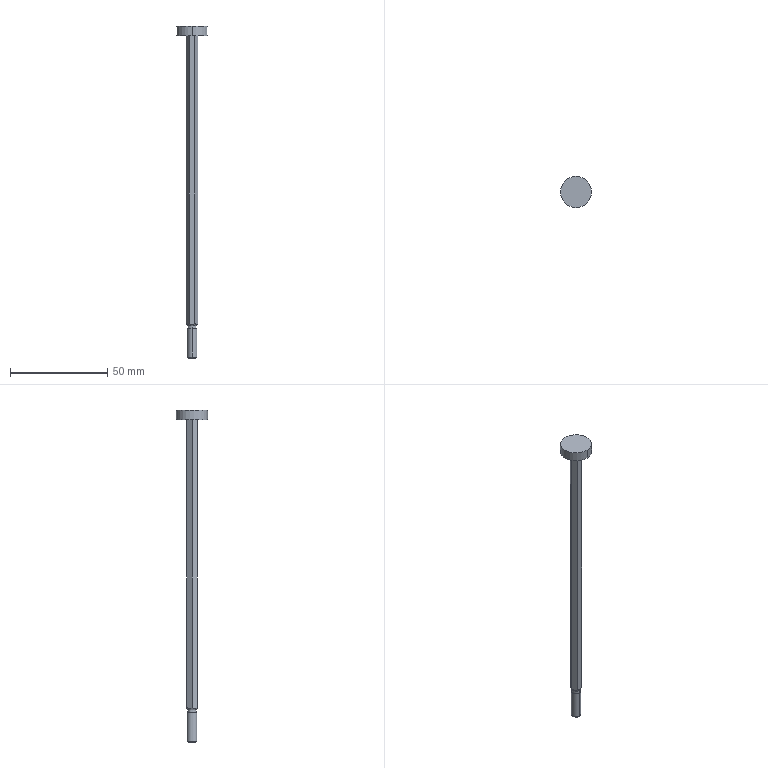Component | SolidWorks | F-YBCJ2RKA16-125_ROD-1 | 1 solid | 20 faces | box 16 x 16 x 170.5 mm | volume 4806 mm3 | plane 10 | cylinder 6 | cone 4 | commonest cylinder face diameters 16 x2 4.43 x2 5 x2
build123d program:
from build123d import *

# Parameters (mm, degrees)
SKETCH2_R          = 5.2
CUT_EXTRUDE1_DEPTH = 150.5


with BuildPart() as part:
    # Sketch1 → Revolve1 (revolve)
    with BuildSketch(Plane.XY, mode=Mode.PRIVATE) as revolve1_sk:
        Polygon((0, 0), (0, 2.01), (0.4905, 2.5), (15, 2.5), (15, 2.215), (16.5, 2.215), (17.864, 3.002), (165.5, 3.002), (165.5, 8), (170.5, 8), (170.5, 0), align=None)
    revolve(revolve1_sk.sketch.rotate(Axis((170.5, 0, 0), (-1, 0, 0)), 180), axis=Axis((170.5, 0, 0), (-1, 0, 0)))

    # Sketch2 → Cut-Extrude1 (cut)
    with BuildSketch(Plane(origin=(15, 0, 0), x_dir=(0, 0, -1), z_dir=(1, 0, 0))):
        Circle(SKETCH2_R)
        Polygon((-3.002, 0), (-1.501, -2.6), (1.501, -2.6), (3.002, 0), (1.501, 2.6), (-1.501, 2.6), align=None, mode=Mode.SUBTRACT)
    extrude(amount=CUT_EXTRUDE1_DEPTH, mode=Mode.SUBTRACT)


solid = part.part

# Placed as in the assembly
solid = solid.moved(Location((272.305, 302.175, 105.479), (0, -90, 0)))
STEP:
#1=COLOUR_RGB('',0.7922,0.8196,0.9333);
#2=FILL_AREA_STYLE_COLOUR('',#1);
#3=FILL_AREA_STYLE('',(#2));
#4=SURFACE_STYLE_FILL_AREA(#3);
#5=SURFACE_SIDE_STYLE('',(#4));
#6=SURFACE_STYLE_USAGE(.BOTH.,#5);
#7=PRESENTATION_STYLE_ASSIGNMENT((#6));
#8=CARTESIAN_POINT('',(10.721,11.582,10.865));
#9=VERTEX_POINT('',#8);
#10=CARTESIAN_POINT('',(10.721,12.212,10.865));
#11=VERTEX_POINT('',#10);
#12=CARTESIAN_POINT('',(10.721,11.897,10.865));
#13=DIRECTION('',(0.,-0.,-1.));
#14=DIRECTION('',(0.,-1.,0.));
#15=AXIS2_PLACEMENT_3D('',#12,#13,#14);
#16=CIRCLE('',#15,0.315);
#17=EDGE_CURVE('',#9,#11,#16,.T.);
#18=ORIENTED_EDGE('',*,*,#17,.T.);
#19=CARTESIAN_POINT('',(10.721,12.212,10.668));
#20=VERTEX_POINT('',#19);
#21=CARTESIAN_POINT('',(10.721,12.212,10.865));
#22=DIRECTION('',(0.,-0.,-1.));
#23=VECTOR('',#22,39.37);
#24=LINE('',#21,#23);
#25=EDGE_CURVE('',#11,#20,#24,.T.);
#26=ORIENTED_EDGE('',*,*,#25,.T.);
#27=CARTESIAN_POINT('',(10.721,11.582,10.668));
#28=VERTEX_POINT('',#27);
#29=CARTESIAN_POINT('',(10.721,11.897,10.668));
#30=DIRECTION('',(0.,-0.,-1.));
#31=DIRECTION('',(0.,-1.,0.));
#32=AXIS2_PLACEMENT_3D('',#29,#30,#31);
#33=CIRCLE('',#32,0.315);
#34=EDGE_CURVE('',#28,#20,#33,.T.);
#35=ORIENTED_EDGE('',*,*,#34,.F.);
#36=CARTESIAN_POINT('',(10.721,11.582,10.865));
#37=DIRECTION('',(0.,-0.,-1.));
#38=VECTOR('',#37,39.37);
#39=LINE('',#36,#38);
#40=EDGE_CURVE('',#9,#28,#39,.T.);
#41=ORIENTED_EDGE('',*,*,#40,.F.);
#42=EDGE_LOOP('',(#18,#26,#35,#41));
#43=FACE_OUTER_BOUND('',#42,.T.);
#44=CARTESIAN_POINT('',(10.721,11.897,10.865));
#45=DIRECTION('',(0.,-0.,-1.));
#46=DIRECTION('',(0.,-1.,0.));
#47=AXIS2_PLACEMENT_3D('',#44,#45,#46);
#48=CYLINDRICAL_SURFACE('',#47,0.315);
#49=ADVANCED_FACE('',(#43),#48,.T.);
#50=CARTESIAN_POINT('',(10.721,11.809,4.802));
#51=VERTEX_POINT('',#50);
#52=CARTESIAN_POINT('',(10.721,11.984,4.802));
#53=VERTEX_POINT('',#52);
#54=CARTESIAN_POINT('',(10.721,11.897,4.802));
#55=DIRECTION('',(0.,-0.,-1.));
#56=DIRECTION('',(0.,-1.,0.));
#57=AXIS2_PLACEMENT_3D('',#54,#55,#56);
#58=CIRCLE('',#57,0.0872);
#59=EDGE_CURVE('',#51,#53,#58,.T.);
#60=ORIENTED_EDGE('',*,*,#59,.F.);
#61=CARTESIAN_POINT('',(10.721,11.794,4.829));
#62=VERTEX_POINT('',#61);
#63=CARTESIAN_POINT('',(10.721,11.778,4.856));
#64=DIRECTION('',(-0.,-0.5,0.866));
#65=VECTOR('',#64,39.37);
#66=LINE('',#63,#65);
#67=EDGE_CURVE('',#51,#62,#66,.T.);
#68=ORIENTED_EDGE('',*,*,#67,.T.);
#69=CARTESIAN_POINT('',(10.662,11.794,4.856));
#70=VERTEX_POINT('',#69);
#71=CARTESIAN_POINT('',(10.721,11.794,4.829));
#72=CARTESIAN_POINT('',(10.71,11.794,4.829));
#73=CARTESIAN_POINT('',(10.699,11.794,4.832));
#74=CARTESIAN_POINT('',(10.679,11.794,4.842));
#75=CARTESIAN_POINT('',(10.67,11.794,4.849));
#76=CARTESIAN_POINT('',(10.662,11.794,4.856));
#77=B_SPLINE_CURVE_WITH_KNOTS('',3,(#71,#72,#73,#74,#75,#76),.UNSPECIFIED.,.F.,.F.,(4,2,4),(0.00333,0.004165,0.005),.UNSPECIFIED.);
#78=EDGE_CURVE('',#62,#70,#77,.T.);
#79=ORIENTED_EDGE('',*,*,#78,.T.);
#80=CARTESIAN_POINT('',(10.602,11.897,4.856));
#81=VERTEX_POINT('',#80);
#82=CARTESIAN_POINT('',(10.662,11.794,4.856));
#83=CARTESIAN_POINT('',(10.657,11.802,4.849));
#84=CARTESIAN_POINT('',(10.653,11.809,4.842));
#85=CARTESIAN_POINT('',(10.646,11.822,4.834));
#86=CARTESIAN_POINT('',(10.643,11.827,4.832));
#87=CARTESIAN_POINT('',(10.638,11.836,4.829));
#88=CARTESIAN_POINT('',(10.635,11.841,4.829));
#89=CARTESIAN_POINT('',(10.627,11.855,4.829));
#90=CARTESIAN_POINT('',(10.621,11.865,4.832));
#91=CARTESIAN_POINT('',(10.611,11.882,4.842));
#92=CARTESIAN_POINT('',(10.607,11.889,4.849));
#93=CARTESIAN_POINT('',(10.602,11.897,4.856));
#94=B_SPLINE_CURVE_WITH_KNOTS('',3,(#82,#83,#84,#85,#86,#87,#88,#89,#90,#91,#92,#93),.UNSPECIFIED.,.F.,.F.,(4,2,2,2,2,4),(0.0000003,0.0008398,0.00126,0.001679,0.002519,0.003358),.UNSPECIFIED.);
#95=EDGE_CURVE('',#70,#81,#94,.T.);
#96=ORIENTED_EDGE('',*,*,#95,.T.);
#97=CARTESIAN_POINT('',(10.662,11.999,4.856));
#98=VERTEX_POINT('',#97);
#99=CARTESIAN_POINT('',(10.602,11.897,4.856));
#100=CARTESIAN_POINT('',(10.607,11.904,4.849));
#101=CARTESIAN_POINT('',(10.611,11.912,4.842));
#102=CARTESIAN_POINT('',(10.618,11.924,4.834));
#103=CARTESIAN_POINT('',(10.621,11.929,4.832));
#104=CARTESIAN_POINT('',(10.626,11.938,4.829));
#105=CARTESIAN_POINT('',(10.629,11.943,4.829));
#106=CARTESIAN_POINT('',(10.638,11.957,4.829));
#107=CARTESIAN_POINT('',(10.643,11.967,4.832));
#108=CARTESIAN_POINT('',(10.653,11.984,4.842));
#109=CARTESIAN_POINT('',(10.657,11.992,4.849));
#110=CARTESIAN_POINT('',(10.662,11.999,4.856));
#111=B_SPLINE_CURVE_WITH_KNOTS('',3,(#99,#100,#101,#102,#103,#104,#105,#106,#107,#108,#109,#110),.UNSPECIFIED.,.F.,.F.,(4,2,2,2,2,4),(0.0000003,0.0008398,0.00126,0.001679,0.002519,0.003358),.UNSPECIFIED.);
#112=EDGE_CURVE('',#81,#98,#111,.T.);
#113=ORIENTED_EDGE('',*,*,#112,.T.);
#114=CARTESIAN_POINT('',(10.721,11.999,4.829));
#115=VERTEX_POINT('',#114);
#116=CARTESIAN_POINT('',(10.662,11.999,4.856));
#117=CARTESIAN_POINT('',(10.67,11.999,4.849));
#118=CARTESIAN_POINT('',(10.679,11.999,4.842));
#119=CARTESIAN_POINT('',(10.699,11.999,4.832));
#120=CARTESIAN_POINT('',(10.71,11.999,4.829));
#121=CARTESIAN_POINT('',(10.721,11.999,4.829));
#122=B_SPLINE_CURVE_WITH_KNOTS('',3,(#116,#117,#118,#119,#120,#121),.UNSPECIFIED.,.F.,.F.,(4,2,4),(0.003237,0.004069,0.004901),.UNSPECIFIED.);
#123=EDGE_CURVE('',#98,#115,#122,.T.);
#124=ORIENTED_EDGE('',*,*,#123,.T.);
#125=CARTESIAN_POINT('',(10.721,12.015,4.856));
#126=DIRECTION('',(-0.,0.5,0.866));
#127=VECTOR('',#126,39.37);
#128=LINE('',#125,#127);
#129=EDGE_CURVE('',#53,#115,#128,.T.);
#130=ORIENTED_EDGE('',*,*,#129,.F.);
#131=EDGE_LOOP('',(#60,#68,#79,#96,#113,#124,#130));
#132=FACE_OUTER_BOUND('',#131,.T.);
#133=CARTESIAN_POINT('',(10.721,11.897,4.856));
#134=DIRECTION('',(-0.,0.,1.));
#135=DIRECTION('',(0.,1.,0.));
#136=AXIS2_PLACEMENT_3D('',#133,#134,#135);
#137=CONICAL_SURFACE('',#136,0.1182,0.5236);
#138=ADVANCED_FACE('',(#132),#137,.T.);
#139=ORIENTED_EDGE('',*,*,#59,.T.);
#140=CARTESIAN_POINT('',(10.721,11.984,4.743));
#141=VERTEX_POINT('',#140);
#142=CARTESIAN_POINT('',(10.721,11.984,10.865));
#143=DIRECTION('',(0.,-0.,-1.));
#144=VECTOR('',#143,39.37);
#145=LINE('',#142,#144);
#146=EDGE_CURVE('',#53,#141,#145,.T.);
#147=ORIENTED_EDGE('',*,*,#146,.T.);
#148=CARTESIAN_POINT('',(10.721,11.809,4.743));
#149=VERTEX_POINT('',#148);
#150=CARTESIAN_POINT('',(10.721,11.897,4.743));
#151=DIRECTION('',(0.,-0.,-1.));
#152=DIRECTION('',(0.,-1.,0.));
#153=AXIS2_PLACEMENT_3D('',#150,#151,#152);
#154=CIRCLE('',#153,0.0872);
#155=EDGE_CURVE('',#149,#141,#154,.T.);
#156=ORIENTED_EDGE('',*,*,#155,.F.);
#157=CARTESIAN_POINT('',(10.721,11.809,10.865));
#158=DIRECTION('',(0.,-0.,-1.));
#159=VECTOR('',#158,39.37);
#160=LINE('',#157,#159);
#161=EDGE_CURVE('',#51,#149,#160,.T.);
#162=ORIENTED_EDGE('',*,*,#161,.F.);
#163=EDGE_LOOP('',(#139,#147,#156,#162));
#164=FACE_OUTER_BOUND('',#163,.T.);
#165=CARTESIAN_POINT('',(10.721,11.897,10.865));
#166=DIRECTION('',(0.,-0.,-1.));
#167=DIRECTION('',(0.,-1.,0.));
#168=AXIS2_PLACEMENT_3D('',#165,#166,#167);
#169=CYLINDRICAL_SURFACE('',#168,0.0872);
#170=ADVANCED_FACE('',(#164),#169,.T.);
#171=CARTESIAN_POINT('',(10.721,11.798,4.743));
#172=VERTEX_POINT('',#171);
#173=CARTESIAN_POINT('',(10.721,11.995,4.743));
#174=VERTEX_POINT('',#173);
#175=CARTESIAN_POINT('',(10.721,11.897,4.743));
#176=DIRECTION('',(0.,-0.,-1.));
#177=DIRECTION('',(0.,-1.,0.));
#178=AXIS2_PLACEMENT_3D('',#175,#176,#177);
#179=CIRCLE('',#178,0.09843);
#180=EDGE_CURVE('',#172,#174,#179,.T.);
#181=ORIENTED_EDGE('',*,*,#180,.T.);
#182=CARTESIAN_POINT('',(10.721,11.995,4.172));
#183=VERTEX_POINT('',#182);
#184=CARTESIAN_POINT('',(10.721,11.995,10.865));
#185=DIRECTION('',(0.,-0.,-1.));
#186=VECTOR('',#185,39.37);
#187=LINE('',#184,#186);
#188=EDGE_CURVE('',#174,#183,#187,.T.);
#189=ORIENTED_EDGE('',*,*,#188,.T.);
#190=CARTESIAN_POINT('',(10.721,11.798,4.172));
#191=VERTEX_POINT('',#190);
#192=CARTESIAN_POINT('',(10.721,11.897,4.172));
#193=DIRECTION('',(0.,-0.,-1.));
#194=DIRECTION('',(0.,-1.,0.));
#195=AXIS2_PLACEMENT_3D('',#192,#193,#194);
#196=CIRCLE('',#195,0.09843);
#197=EDGE_CURVE('',#191,#183,#196,.T.);
#198=ORIENTED_EDGE('',*,*,#197,.F.);
#199=CARTESIAN_POINT('',(10.721,11.798,10.865));
#200=DIRECTION('',(0.,-0.,-1.));
#201=VECTOR('',#200,39.37);
#202=LINE('',#199,#201);
#203=EDGE_CURVE('',#172,#191,#202,.T.);
#204=ORIENTED_EDGE('',*,*,#203,.F.);
#205=EDGE_LOOP('',(#181,#189,#198,#204));
#206=FACE_OUTER_BOUND('',#205,.T.);
#207=CARTESIAN_POINT('',(10.721,11.897,10.865));
#208=DIRECTION('',(0.,-0.,-1.));
#209=DIRECTION('',(0.,-1.,0.));
#210=AXIS2_PLACEMENT_3D('',#207,#208,#209);
#211=CYLINDRICAL_SURFACE('',#210,0.09843);
#212=ADVANCED_FACE('',(#206),#211,.T.);
#213=CARTESIAN_POINT('',(10.721,11.818,4.153));
#214=VERTEX_POINT('',#213);
#215=CARTESIAN_POINT('',(10.721,11.976,4.153));
#216=VERTEX_POINT('',#215);
#217=CARTESIAN_POINT('',(10.721,11.897,4.153));
#218=DIRECTION('',(0.,-0.,-1.));
#219=DIRECTION('',(0.,-1.,0.));
#220=AXIS2_PLACEMENT_3D('',#217,#218,#219);
#221=CIRCLE('',#220,0.07911);
#222=EDGE_CURVE('',#214,#216,#221,.T.);
#223=ORIENTED_EDGE('',*,*,#222,.F.);
#224=CARTESIAN_POINT('',(10.721,11.798,4.172));
#225=DIRECTION('',(-0.,-0.7071,0.7071));
#226=VECTOR('',#225,39.37);
#227=LINE('',#224,#226);
#228=EDGE_CURVE('',#214,#191,#227,.T.);
#229=ORIENTED_EDGE('',*,*,#228,.T.);
#230=ORIENTED_EDGE('',*,*,#197,.T.);
#231=CARTESIAN_POINT('',(10.721,11.995,4.172));
#232=DIRECTION('',(-0.,0.7071,0.7071));
#233=VECTOR('',#232,39.37);
#234=LINE('',#231,#233);
#235=EDGE_CURVE('',#216,#183,#234,.T.);
#236=ORIENTED_EDGE('',*,*,#235,.F.);
#237=EDGE_LOOP('',(#223,#229,#230,#236));
#238=FACE_OUTER_BOUND('',#237,.T.);
#239=CARTESIAN_POINT('',(10.721,11.897,4.172));
#240=DIRECTION('',(-0.,0.,1.));
#241=DIRECTION('',(0.,1.,0.));
#242=AXIS2_PLACEMENT_3D('',#239,#240,#241);
#243=CONICAL_SURFACE('',#242,0.09843,0.7854);
#244=ADVANCED_FACE('',(#238),#243,.T.);
#245=CARTESIAN_POINT('',(10.721,11.897,4.153));
#246=DIRECTION('',(0.,-0.,-1.));
#247=DIRECTION('',(0.,-1.,0.));
#248=AXIS2_PLACEMENT_3D('',#245,#246,#247);
#249=CIRCLE('',#248,0.07911);
#250=EDGE_CURVE('',#216,#214,#249,.T.);
#251=ORIENTED_EDGE('',*,*,#250,.T.);
#252=ORIENTED_EDGE('',*,*,#222,.T.);
#253=EDGE_LOOP('',(#251,#252));
#254=FACE_OUTER_BOUND('',#253,.T.);
#255=CARTESIAN_POINT('',(10.721,11.897,4.153));
#256=DIRECTION('',(-0.,0.,1.));
#257=DIRECTION('',(0.,1.,-0.));
#258=AXIS2_PLACEMENT_3D('',#255,#256,#257);
#259=PLANE('',#258);
#260=ADVANCED_FACE('',(#254),#259,.F.);
#261=ORIENTED_EDGE('',*,*,#228,.F.);
#262=ORIENTED_EDGE('',*,*,#250,.F.);
#263=ORIENTED_EDGE('',*,*,#235,.T.);
#264=CARTESIAN_POINT('',(10.721,11.897,4.172));
#265=DIRECTION('',(0.,-0.,-1.));
#266=DIRECTION('',(0.,-1.,0.));
#267=AXIS2_PLACEMENT_3D('',#264,#265,#266);
#268=CIRCLE('',#267,0.09843);
#269=EDGE_CURVE('',#183,#191,#268,.T.);
#270=ORIENTED_EDGE('',*,*,#269,.T.);
#271=EDGE_LOOP('',(#261,#262,#263,#270));
#272=FACE_OUTER_BOUND('',#271,.T.);
#273=CARTESIAN_POINT('',(10.721,11.897,4.172));
#274=DIRECTION('',(-0.,0.,1.));
#275=DIRECTION('',(0.,1.,0.));
#276=AXIS2_PLACEMENT_3D('',#273,#274,#275);
#277=CONICAL_SURFACE('',#276,0.09843,0.7854);
#278=ADVANCED_FACE('',(#272),#277,.T.);
#279=ORIENTED_EDGE('',*,*,#188,.F.);
#280=CARTESIAN_POINT('',(10.721,11.897,4.743));
#281=DIRECTION('',(0.,-0.,-1.));
#282=DIRECTION('',(0.,-1.,0.));
#283=AXIS2_PLACEMENT_3D('',#280,#281,#282);
#284=CIRCLE('',#283,0.09843);
#285=EDGE_CURVE('',#174,#172,#284,.T.);
#286=ORIENTED_EDGE('',*,*,#285,.T.);
#287=ORIENTED_EDGE('',*,*,#203,.T.);
#288=ORIENTED_EDGE('',*,*,#269,.F.);
#289=EDGE_LOOP('',(#279,#286,#287,#288));
#290=FACE_OUTER_BOUND('',#289,.T.);
#291=CARTESIAN_POINT('',(10.721,11.897,10.865));
#292=DIRECTION('',(0.,-0.,-1.));
#293=DIRECTION('',(0.,-1.,0.));
#294=AXIS2_PLACEMENT_3D('',#291,#292,#293);
#295=CYLINDRICAL_SURFACE('',#294,0.09843);
#296=ADVANCED_FACE('',(#290),#295,.T.);
#297=ORIENTED_EDGE('',*,*,#180,.F.);
#298=ORIENTED_EDGE('',*,*,#285,.F.);
#299=EDGE_LOOP('',(#297,#298));
#300=FACE_OUTER_BOUND('',#299,.T.);
#301=ORIENTED_EDGE('',*,*,#155,.T.);
#302=CARTESIAN_POINT('',(10.721,11.897,4.743));
#303=DIRECTION('',(0.,-0.,-1.));
#304=DIRECTION('',(0.,-1.,0.));
#305=AXIS2_PLACEMENT_3D('',#302,#303,#304);
#306=CIRCLE('',#305,0.0872);
#307=EDGE_CURVE('',#141,#149,#306,.T.);
#308=ORIENTED_EDGE('',*,*,#307,.T.);
#309=EDGE_LOOP('',(#301,#308));
#310=FACE_BOUND('',#309,.T.);
#311=CARTESIAN_POINT('',(10.721,11.995,4.743));
#312=DIRECTION('',(0.,-0.,-1.));
#313=DIRECTION('',(-0.,-1.,0.));
#314=AXIS2_PLACEMENT_3D('',#311,#312,#313);
#315=PLANE('',#314);
#316=ADVANCED_FACE('',(#300,#310),#315,.F.);
#317=ORIENTED_EDGE('',*,*,#146,.F.);
#318=CARTESIAN_POINT('',(10.721,11.897,4.802));
#319=DIRECTION('',(0.,-0.,-1.));
#320=DIRECTION('',(0.,-1.,0.));
#321=AXIS2_PLACEMENT_3D('',#318,#319,#320);
#322=CIRCLE('',#321,0.0872);
#323=EDGE_CURVE('',#53,#51,#322,.T.);
#324=ORIENTED_EDGE('',*,*,#323,.T.);
#325=ORIENTED_EDGE('',*,*,#161,.T.);
#326=ORIENTED_EDGE('',*,*,#307,.F.);
#327=EDGE_LOOP('',(#317,#324,#325,#326));
#328=FACE_OUTER_BOUND('',#327,.T.);
#329=CARTESIAN_POINT('',(10.721,11.897,10.865));
#330=DIRECTION('',(0.,-0.,-1.));
#331=DIRECTION('',(0.,-1.,0.));
#332=AXIS2_PLACEMENT_3D('',#329,#330,#331);
#333=CYLINDRICAL_SURFACE('',#332,0.0872);
#334=ADVANCED_FACE('',(#328),#333,.T.);
#335=ORIENTED_EDGE('',*,*,#67,.F.);
#336=ORIENTED_EDGE('',*,*,#323,.F.);
#337=ORIENTED_EDGE('',*,*,#129,.T.);
#338=CARTESIAN_POINT('',(10.78,11.999,4.856));
#339=VERTEX_POINT('',#338);
#340=CARTESIAN_POINT('',(10.721,11.999,4.829));
#341=CARTESIAN_POINT('',(10.732,11.999,4.829));
#342=CARTESIAN_POINT('',(10.743,11.999,4.832));
#343=CARTESIAN_POINT('',(10.762,11.999,4.842));
#344=CARTESIAN_POINT('',(10.771,11.999,4.849));
#345=CARTESIAN_POINT('',(10.78,11.999,4.856));
#346=B_SPLINE_CURVE_WITH_KNOTS('',3,(#340,#341,#342,#343,#344,#345),.UNSPECIFIED.,.F.,.F.,(4,2,4),(0.004901,0.005734,0.006567),.UNSPECIFIED.);
#347=EDGE_CURVE('',#115,#339,#346,.T.);
#348=ORIENTED_EDGE('',*,*,#347,.T.);
#349=CARTESIAN_POINT('',(10.839,11.897,4.856));
#350=VERTEX_POINT('',#349);
#351=CARTESIAN_POINT('',(10.78,11.999,4.856));
#352=CARTESIAN_POINT('',(10.784,11.992,4.849));
#353=CARTESIAN_POINT('',(10.788,11.984,4.842));
#354=CARTESIAN_POINT('',(10.796,11.971,4.834));
#355=CARTESIAN_POINT('',(10.798,11.967,4.832));
#356=CARTESIAN_POINT('',(10.804,11.958,4.829));
#357=CARTESIAN_POINT('',(10.807,11.953,4.829));
#358=CARTESIAN_POINT('',(10.815,11.938,4.829));
#359=CARTESIAN_POINT('',(10.82,11.929,4.832));
#360=CARTESIAN_POINT('',(10.83,11.912,4.842));
#361=CARTESIAN_POINT('',(10.835,11.904,4.849));
#362=CARTESIAN_POINT('',(10.839,11.897,4.856));
#363=B_SPLINE_CURVE_WITH_KNOTS('',3,(#351,#352,#353,#354,#355,#356,#357,#358,#359,#360,#361,#362),.UNSPECIFIED.,.F.,.F.,(4,2,2,2,2,4),(0.0000003,0.0008398,0.00126,0.001679,0.002519,0.003358),.UNSPECIFIED.);
#364=EDGE_CURVE('',#339,#350,#363,.T.);
#365=ORIENTED_EDGE('',*,*,#364,.T.);
#366=CARTESIAN_POINT('',(10.78,11.794,4.856));
#367=VERTEX_POINT('',#366);
#368=CARTESIAN_POINT('',(10.839,11.897,4.856));
#369=CARTESIAN_POINT('',(10.835,11.889,4.849));
#370=CARTESIAN_POINT('',(10.83,11.882,4.842));
#371=CARTESIAN_POINT('',(10.823,11.869,4.834));
#372=CARTESIAN_POINT('',(10.82,11.864,4.832));
#373=CARTESIAN_POINT('',(10.815,11.855,4.829));
#374=CARTESIAN_POINT('',(10.812,11.85,4.829));
#375=CARTESIAN_POINT('',(10.804,11.836,4.829));
#376=CARTESIAN_POINT('',(10.798,11.826,4.832));
#377=CARTESIAN_POINT('',(10.789,11.809,4.842));
#378=CARTESIAN_POINT('',(10.784,11.802,4.849));
#379=CARTESIAN_POINT('',(10.78,11.794,4.856));
#380=B_SPLINE_CURVE_WITH_KNOTS('',3,(#368,#369,#370,#371,#372,#373,#374,#375,#376,#377,#378,#379),.UNSPECIFIED.,.F.,.F.,(4,2,2,2,2,4),(0.0000003,0.0008398,0.00126,0.001679,0.002519,0.003358),.UNSPECIFIED.);
#381=EDGE_CURVE('',#350,#367,#380,.T.);
#382=ORIENTED_EDGE('',*,*,#381,.T.);
#383=CARTESIAN_POINT('',(10.78,11.794,4.856));
#384=CARTESIAN_POINT('',(10.771,11.794,4.849));
#385=CARTESIAN_POINT('',(10.762,11.794,4.842));
#386=CARTESIAN_POINT('',(10.743,11.794,4.832));
#387=CARTESIAN_POINT('',(10.732,11.794,4.829));
#388=CARTESIAN_POINT('',(10.721,11.794,4.829));
#389=B_SPLINE_CURVE_WITH_KNOTS('',3,(#383,#384,#385,#386,#387,#388),.UNSPECIFIED.,.F.,.F.,(4,2,4),(0.001658,0.002494,0.00333),.UNSPECIFIED.);
#390=EDGE_CURVE('',#367,#62,#389,.T.);
#391=ORIENTED_EDGE('',*,*,#390,.T.);
#392=EDGE_LOOP('',(#335,#336,#337,#348,#365,#382,#391));
#393=FACE_OUTER_BOUND('',#392,.T.);
#394=CARTESIAN_POINT('',(10.721,11.897,4.856));
#395=DIRECTION('',(-0.,0.,1.));
#396=DIRECTION('',(0.,1.,0.));
#397=AXIS2_PLACEMENT_3D('',#394,#395,#396);
#398=CONICAL_SURFACE('',#397,0.1182,0.5236);
#399=ADVANCED_FACE('',(#393),#398,.T.);
#400=CARTESIAN_POINT('',(10.602,11.897,10.668));
#401=VERTEX_POINT('',#400);
#402=CARTESIAN_POINT('',(10.602,11.897,10.668));
#403=DIRECTION('',(0.,0.,-1.));
#404=VECTOR('',#403,39.37);
#405=LINE('',#402,#404);
#406=EDGE_CURVE('',#401,#81,#405,.T.);
#407=ORIENTED_EDGE('',*,*,#406,.F.);
#408=CARTESIAN_POINT('',(10.662,11.999,10.668));
#409=VERTEX_POINT('',#408);
#410=CARTESIAN_POINT('',(10.662,11.999,10.668));
#411=DIRECTION('',(-0.5,-0.866,-0.));
#412=VECTOR('',#411,39.37);
#413=LINE('',#410,#412);
#414=EDGE_CURVE('',#409,#401,#413,.T.);
#415=ORIENTED_EDGE('',*,*,#414,.F.);
#416=CARTESIAN_POINT('',(10.662,11.999,10.668));
#417=DIRECTION('',(0.,0.,-1.));
#418=VECTOR('',#417,39.37);
#419=LINE('',#416,#418);
#420=EDGE_CURVE('',#409,#98,#419,.T.);
#421=ORIENTED_EDGE('',*,*,#420,.T.);
#422=ORIENTED_EDGE('',*,*,#112,.F.);
#423=EDGE_LOOP('',(#407,#415,#421,#422));
#424=FACE_OUTER_BOUND('',#423,.T.);
#425=CARTESIAN_POINT('',(10.662,11.999,10.668));
#426=DIRECTION('',(0.866,-0.5,0.));
#427=DIRECTION('',(0.5,0.866,0.));
#428=AXIS2_PLACEMENT_3D('',#425,#426,#427);
#429=PLANE('',#428);
#430=ADVANCED_FACE('',(#424),#429,.F.);
#431=CARTESIAN_POINT('',(10.662,11.794,10.668));
#432=VERTEX_POINT('',#431);
#433=CARTESIAN_POINT('',(10.662,11.794,10.668));
#434=DIRECTION('',(0.,0.,-1.));
#435=VECTOR('',#434,39.37);
#436=LINE('',#433,#435);
#437=EDGE_CURVE('',#432,#70,#436,.T.);
#438=ORIENTED_EDGE('',*,*,#437,.F.);
#439=CARTESIAN_POINT('',(10.602,11.897,10.668));
#440=DIRECTION('',(0.5,-0.866,0.));
#441=VECTOR('',#440,39.37);
#442=LINE('',#439,#441);
#443=EDGE_CURVE('',#401,#432,#442,.T.);
#444=ORIENTED_EDGE('',*,*,#443,.F.);
#445=ORIENTED_EDGE('',*,*,#406,.T.);
#446=ORIENTED_EDGE('',*,*,#95,.F.);
#447=EDGE_LOOP('',(#438,#444,#445,#446));
#448=FACE_OUTER_BOUND('',#447,.T.);
#449=CARTESIAN_POINT('',(10.602,11.897,10.668));
#450=DIRECTION('',(0.866,0.5,0.));
#451=DIRECTION('',(-0.5,0.866,-0.));
#452=AXIS2_PLACEMENT_3D('',#449,#450,#451);
#453=PLANE('',#452);
#454=ADVANCED_FACE('',(#448),#453,.F.);
#455=CARTESIAN_POINT('',(10.78,11.794,10.668));
#456=VERTEX_POINT('',#455);
#457=CARTESIAN_POINT('',(10.78,11.794,10.668));
#458=DIRECTION('',(0.,0.,-1.));
#459=VECTOR('',#458,39.37);
#460=LINE('',#457,#459);
#461=EDGE_CURVE('',#456,#367,#460,.T.);
#462=ORIENTED_EDGE('',*,*,#461,.F.);
#463=CARTESIAN_POINT('',(10.662,11.794,10.668));
#464=DIRECTION('',(1.,-0.,0.));
#465=VECTOR('',#464,39.37);
#466=LINE('',#463,#465);
#467=EDGE_CURVE('',#432,#456,#466,.T.);
#468=ORIENTED_EDGE('',*,*,#467,.F.);
#469=ORIENTED_EDGE('',*,*,#437,.T.);
#470=ORIENTED_EDGE('',*,*,#78,.F.);
#471=ORIENTED_EDGE('',*,*,#390,.F.);
#472=EDGE_LOOP('',(#462,#468,#469,#470,#471));
#473=FACE_OUTER_BOUND('',#472,.T.);
#474=CARTESIAN_POINT('',(10.662,11.794,10.668));
#475=DIRECTION('',(0.,1.,0.));
#476=DIRECTION('',(-1.,0.,-0.));
#477=AXIS2_PLACEMENT_3D('',#474,#475,#476);
#478=PLANE('',#477);
#479=ADVANCED_FACE('',(#473),#478,.F.);
#480=CARTESIAN_POINT('',(10.839,11.897,10.668));
#481=VERTEX_POINT('',#480);
#482=CARTESIAN_POINT('',(10.839,11.897,10.668));
#483=DIRECTION('',(0.,0.,-1.));
#484=VECTOR('',#483,39.37);
#485=LINE('',#482,#484);
#486=EDGE_CURVE('',#481,#350,#485,.T.);
#487=ORIENTED_EDGE('',*,*,#486,.F.);
#488=CARTESIAN_POINT('',(10.78,11.794,10.668));
#489=DIRECTION('',(0.5,0.866,0.));
#490=VECTOR('',#489,39.37);
#491=LINE('',#488,#490);
#492=EDGE_CURVE('',#456,#481,#491,.T.);
#493=ORIENTED_EDGE('',*,*,#492,.F.);
#494=ORIENTED_EDGE('',*,*,#461,.T.);
#495=ORIENTED_EDGE('',*,*,#381,.F.);
#496=EDGE_LOOP('',(#487,#493,#494,#495));
#497=FACE_OUTER_BOUND('',#496,.T.);
#498=CARTESIAN_POINT('',(10.78,11.794,10.668));
#499=DIRECTION('',(-0.866,0.5,-0.));
#500=DIRECTION('',(-0.5,-0.866,-0.));
#501=AXIS2_PLACEMENT_3D('',#498,#499,#500);
#502=PLANE('',#501);
#503=ADVANCED_FACE('',(#497),#502,.F.);
#504=CARTESIAN_POINT('',(10.78,11.999,10.668));
#505=VERTEX_POINT('',#504);
#506=CARTESIAN_POINT('',(10.78,11.999,10.668));
#507=DIRECTION('',(0.,0.,-1.));
#508=VECTOR('',#507,39.37);
#509=LINE('',#506,#508);
#510=EDGE_CURVE('',#505,#339,#509,.T.);
#511=ORIENTED_EDGE('',*,*,#510,.F.);
#512=CARTESIAN_POINT('',(10.839,11.897,10.668));
#513=DIRECTION('',(-0.5,0.866,-0.));
#514=VECTOR('',#513,39.37);
#515=LINE('',#512,#514);
#516=EDGE_CURVE('',#481,#505,#515,.T.);
#517=ORIENTED_EDGE('',*,*,#516,.F.);
#518=ORIENTED_EDGE('',*,*,#486,.T.);
#519=ORIENTED_EDGE('',*,*,#364,.F.);
#520=EDGE_LOOP('',(#511,#517,#518,#519));
#521=FACE_OUTER_BOUND('',#520,.T.);
#522=CARTESIAN_POINT('',(10.839,11.897,10.668));
#523=DIRECTION('',(-0.866,-0.5,-0.));
#524=DIRECTION('',(0.5,-0.866,0.));
#525=AXIS2_PLACEMENT_3D('',#522,#523,#524);
#526=PLANE('',#525);
#527=ADVANCED_FACE('',(#521),#526,.F.);
#528=ORIENTED_EDGE('',*,*,#420,.F.);
#529=CARTESIAN_POINT('',(10.78,11.999,10.668));
#530=DIRECTION('',(-1.,0.,-0.));
#531=VECTOR('',#530,39.37);
#532=LINE('',#529,#531);
#533=EDGE_CURVE('',#505,#409,#532,.T.);
#534=ORIENTED_EDGE('',*,*,#533,.F.);
#535=ORIENTED_EDGE('',*,*,#510,.T.);
#536=ORIENTED_EDGE('',*,*,#347,.F.);
#537=ORIENTED_EDGE('',*,*,#123,.F.);
#538=EDGE_LOOP('',(#528,#534,#535,#536,#537));
#539=FACE_OUTER_BOUND('',#538,.T.);
#540=CARTESIAN_POINT('',(10.78,11.999,10.668));
#541=DIRECTION('',(-0.,-1.,-0.));
#542=DIRECTION('',(1.,-0.,0.));
#543=AXIS2_PLACEMENT_3D('',#540,#541,#542);
#544=PLANE('',#543);
#545=ADVANCED_FACE('',(#539),#544,.F.);
#546=ORIENTED_EDGE('',*,*,#17,.F.);
#547=CARTESIAN_POINT('',(10.721,11.897,10.865));
#548=DIRECTION('',(0.,-0.,-1.));
#549=DIRECTION('',(0.,-1.,0.));
#550=AXIS2_PLACEMENT_3D('',#547,#548,#549);
#551=CIRCLE('',#550,0.315);
#552=EDGE_CURVE('',#11,#9,#551,.T.);
#553=ORIENTED_EDGE('',*,*,#552,.F.);
#554=EDGE_LOOP('',(#546,#553));
#555=FACE_OUTER_BOUND('',#554,.T.);
#556=CARTESIAN_POINT('',(10.721,12.212,10.865));
#557=DIRECTION('',(0.,-0.,-1.));
#558=DIRECTION('',(-0.,-1.,0.));
#559=AXIS2_PLACEMENT_3D('',#556,#557,#558);
#560=PLANE('',#559);
#561=ADVANCED_FACE('',(#555),#560,.F.);
#562=ORIENTED_EDGE('',*,*,#25,.F.);
#563=ORIENTED_EDGE('',*,*,#552,.T.);
#564=ORIENTED_EDGE('',*,*,#40,.T.);
#565=CARTESIAN_POINT('',(10.721,11.897,10.668));
#566=DIRECTION('',(0.,-0.,-1.));
#567=DIRECTION('',(0.,-1.,0.));
#568=AXIS2_PLACEMENT_3D('',#565,#566,#567);
#569=CIRCLE('',#568,0.315);
#570=EDGE_CURVE('',#20,#28,#569,.T.);
#571=ORIENTED_EDGE('',*,*,#570,.F.);
#572=EDGE_LOOP('',(#562,#563,#564,#571));
#573=FACE_OUTER_BOUND('',#572,.T.);
#574=CARTESIAN_POINT('',(10.721,11.897,10.865));
#575=DIRECTION('',(0.,-0.,-1.));
#576=DIRECTION('',(0.,-1.,0.));
#577=AXIS2_PLACEMENT_3D('',#574,#575,#576);
#578=CYLINDRICAL_SURFACE('',#577,0.315);
#579=ADVANCED_FACE('',(#573),#578,.T.);
#580=ORIENTED_EDGE('',*,*,#492,.T.);
#581=ORIENTED_EDGE('',*,*,#516,.T.);
#582=ORIENTED_EDGE('',*,*,#533,.T.);
#583=ORIENTED_EDGE('',*,*,#414,.T.);
#584=ORIENTED_EDGE('',*,*,#443,.T.);
#585=ORIENTED_EDGE('',*,*,#467,.T.);
#586=EDGE_LOOP('',(#580,#581,#582,#583,#584,#585));
#587=FACE_BOUND('',#586,.T.);
#588=ORIENTED_EDGE('',*,*,#34,.T.);
#589=ORIENTED_EDGE('',*,*,#570,.T.);
#590=EDGE_LOOP('',(#588,#589));
#591=FACE_OUTER_BOUND('',#590,.T.);
#592=CARTESIAN_POINT('',(10.721,12.015,10.668));
#593=DIRECTION('',(-0.,0.,1.));
#594=DIRECTION('',(0.,1.,-0.));
#595=AXIS2_PLACEMENT_3D('',#592,#593,#594);
#596=PLANE('',#595);
#597=ADVANCED_FACE('',(#587,#591),#596,.F.);
#598=CLOSED_SHELL('',(#49,#138,#170,#212,#244,#260,#278,#296,#316,#334,#399,#430,#454,#479,#503,#527,#545,#561,#579,#597));
#599=MANIFOLD_SOLID_BREP('',#598);
#600=STYLED_ITEM('',(#7),#599);
#601=(LENGTH_UNIT()NAMED_UNIT(*)SI_UNIT($,.METRE.));
#602=LENGTH_MEASURE_WITH_UNIT(LENGTH_MEASURE(0.0254),#601);
#603=DIMENSIONAL_EXPONENTS(1.,0.,0.,0.,0.,0.,0.);
#604=(CONVERSION_BASED_UNIT('',#602)LENGTH_UNIT()NAMED_UNIT(#603));
#605=UNCERTAINTY_MEASURE_WITH_UNIT(LENGTH_MEASURE(0.00001),#604,'','');
#606=(NAMED_UNIT(*)PLANE_ANGLE_UNIT()SI_UNIT($,.RADIAN.));
#607=(NAMED_UNIT(*)SI_UNIT($,.STERADIAN.)SOLID_ANGLE_UNIT());
#608=(GEOMETRIC_REPRESENTATION_CONTEXT(3)GLOBAL_UNCERTAINTY_ASSIGNED_CONTEXT((#605))GLOBAL_UNIT_ASSIGNED_CONTEXT((#604,#606,#607))REPRESENTATION_CONTEXT('',''));
#609=MECHANICAL_DESIGN_GEOMETRIC_PRESENTATION_REPRESENTATION('',(#600),#608);
#610=CARTESIAN_POINT('',(0.,0.,0.));
#611=DIRECTION('',(0.,0.,1.));
#612=DIRECTION('',(1.,0.,0.));
#613=AXIS2_PLACEMENT_3D('',#610,#611,#612);
#614=(LENGTH_UNIT()NAMED_UNIT(*)SI_UNIT($,.METRE.));
#615=LENGTH_MEASURE_WITH_UNIT(LENGTH_MEASURE(0.0254),#614);
#616=DIMENSIONAL_EXPONENTS(1.,0.,0.,0.,0.,0.,0.);
#617=(CONVERSION_BASED_UNIT('',#615)LENGTH_UNIT()NAMED_UNIT(#616));
#618=UNCERTAINTY_MEASURE_WITH_UNIT(LENGTH_MEASURE(0.00001),#617,'','');
#619=(NAMED_UNIT(*)PLANE_ANGLE_UNIT()SI_UNIT($,.RADIAN.));
#620=(NAMED_UNIT(*)SI_UNIT($,.STERADIAN.)SOLID_ANGLE_UNIT());
#621=(GEOMETRIC_REPRESENTATION_CONTEXT(3)GLOBAL_UNCERTAINTY_ASSIGNED_CONTEXT((#618))GLOBAL_UNIT_ASSIGNED_CONTEXT((#617,#619,#620))REPRESENTATION_CONTEXT('',''));
#622=ADVANCED_BREP_SHAPE_REPRESENTATION('',(#599,#613),#621);
#623=PRESENTATION_LAYER_ASSIGNMENT('','',(#600));